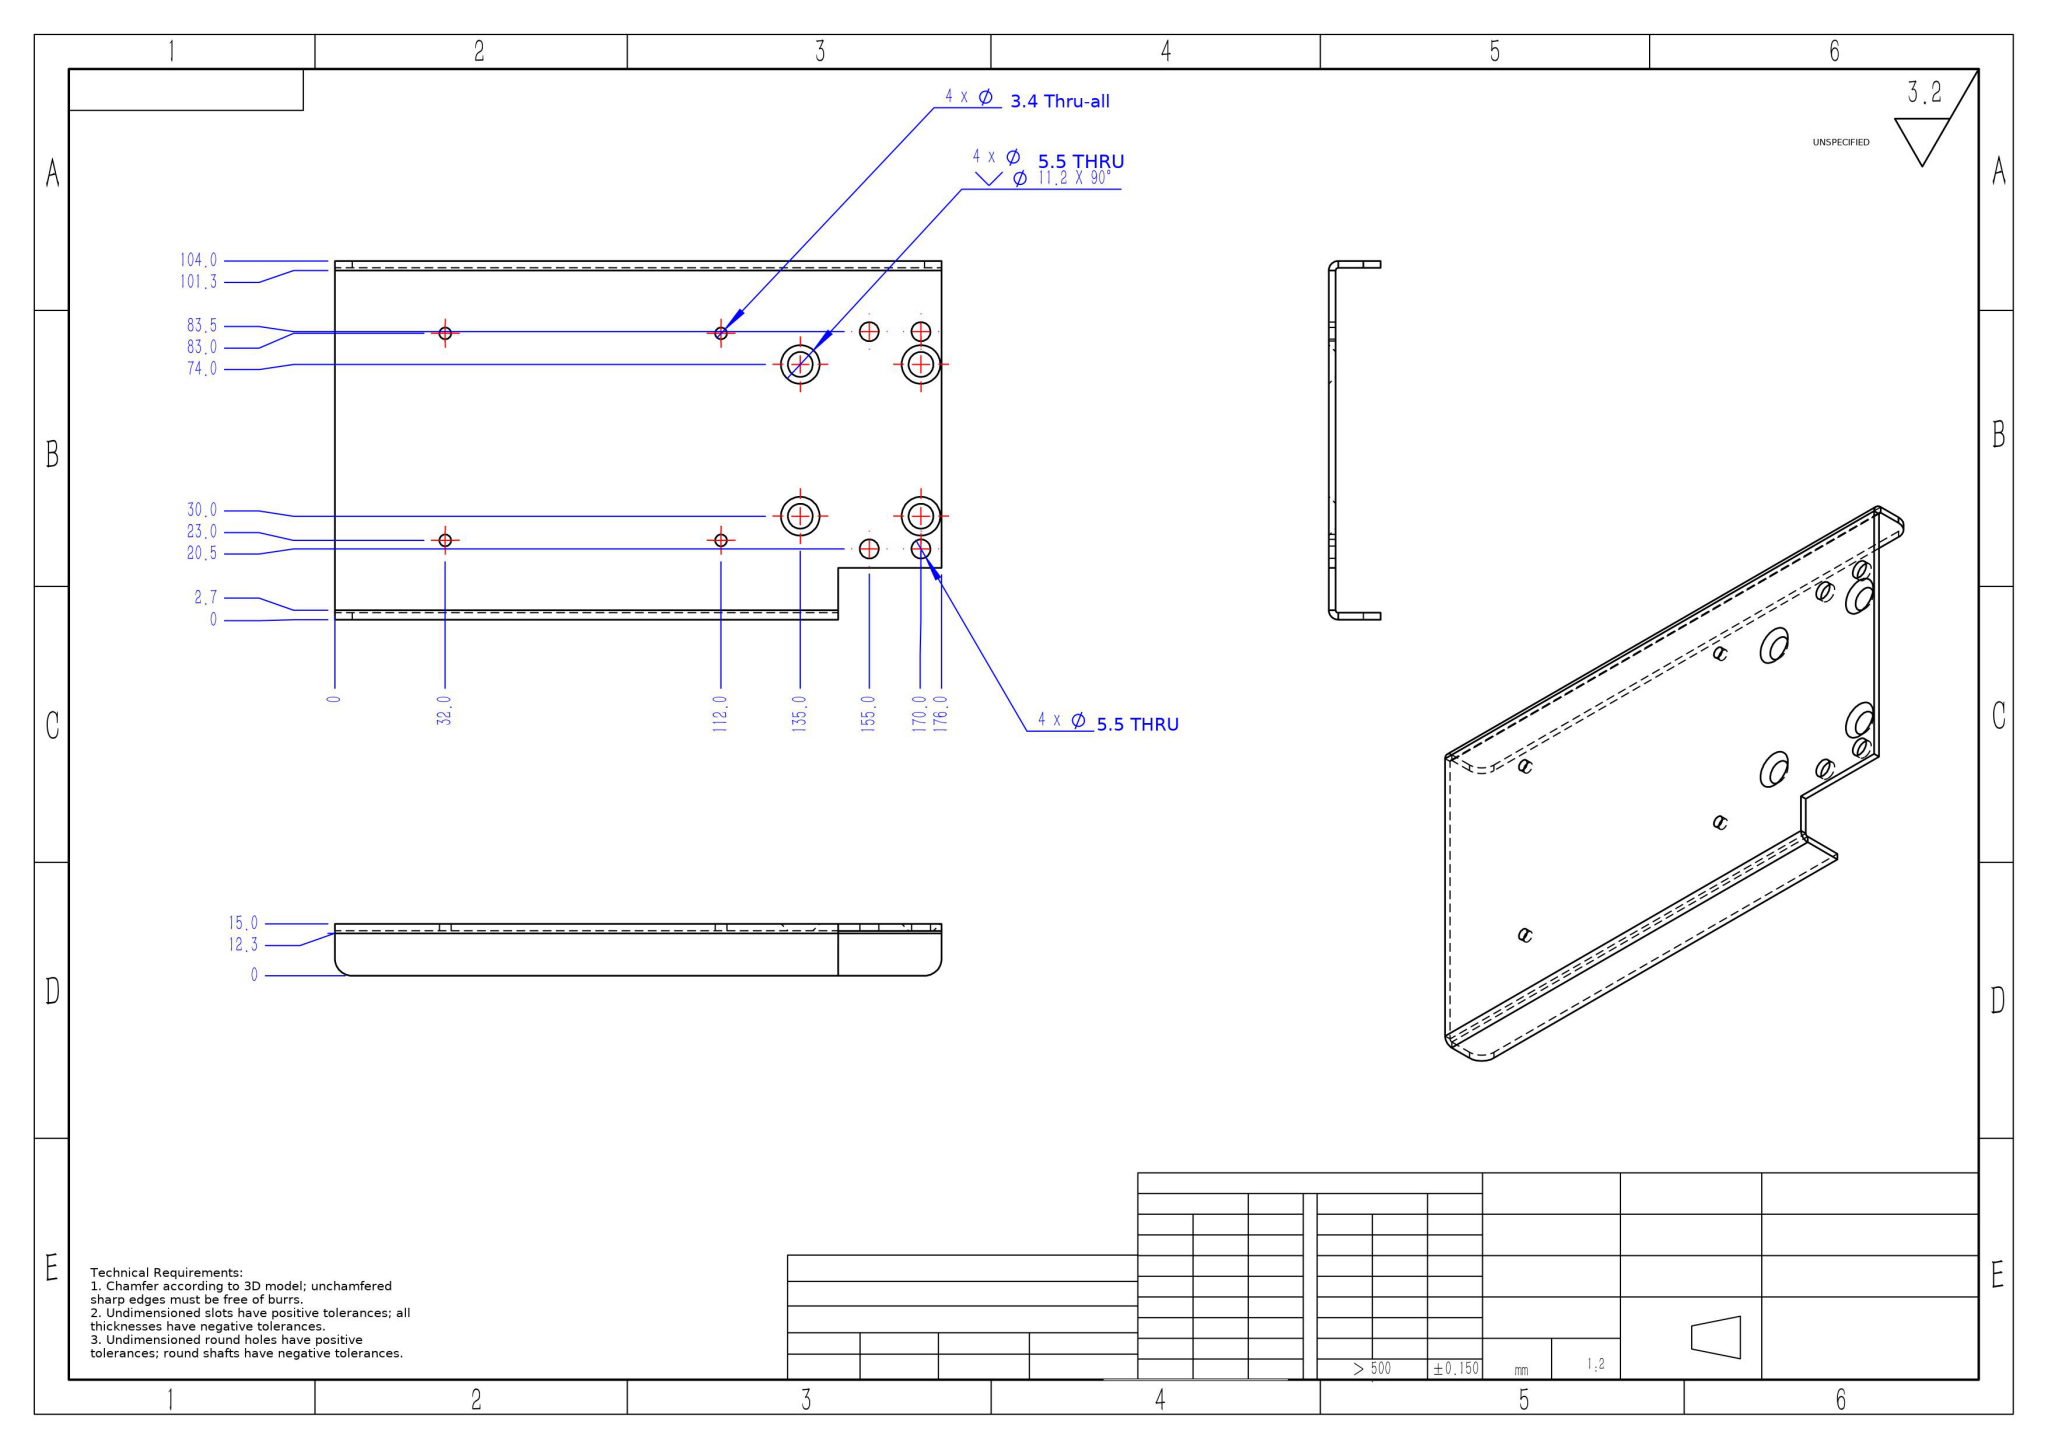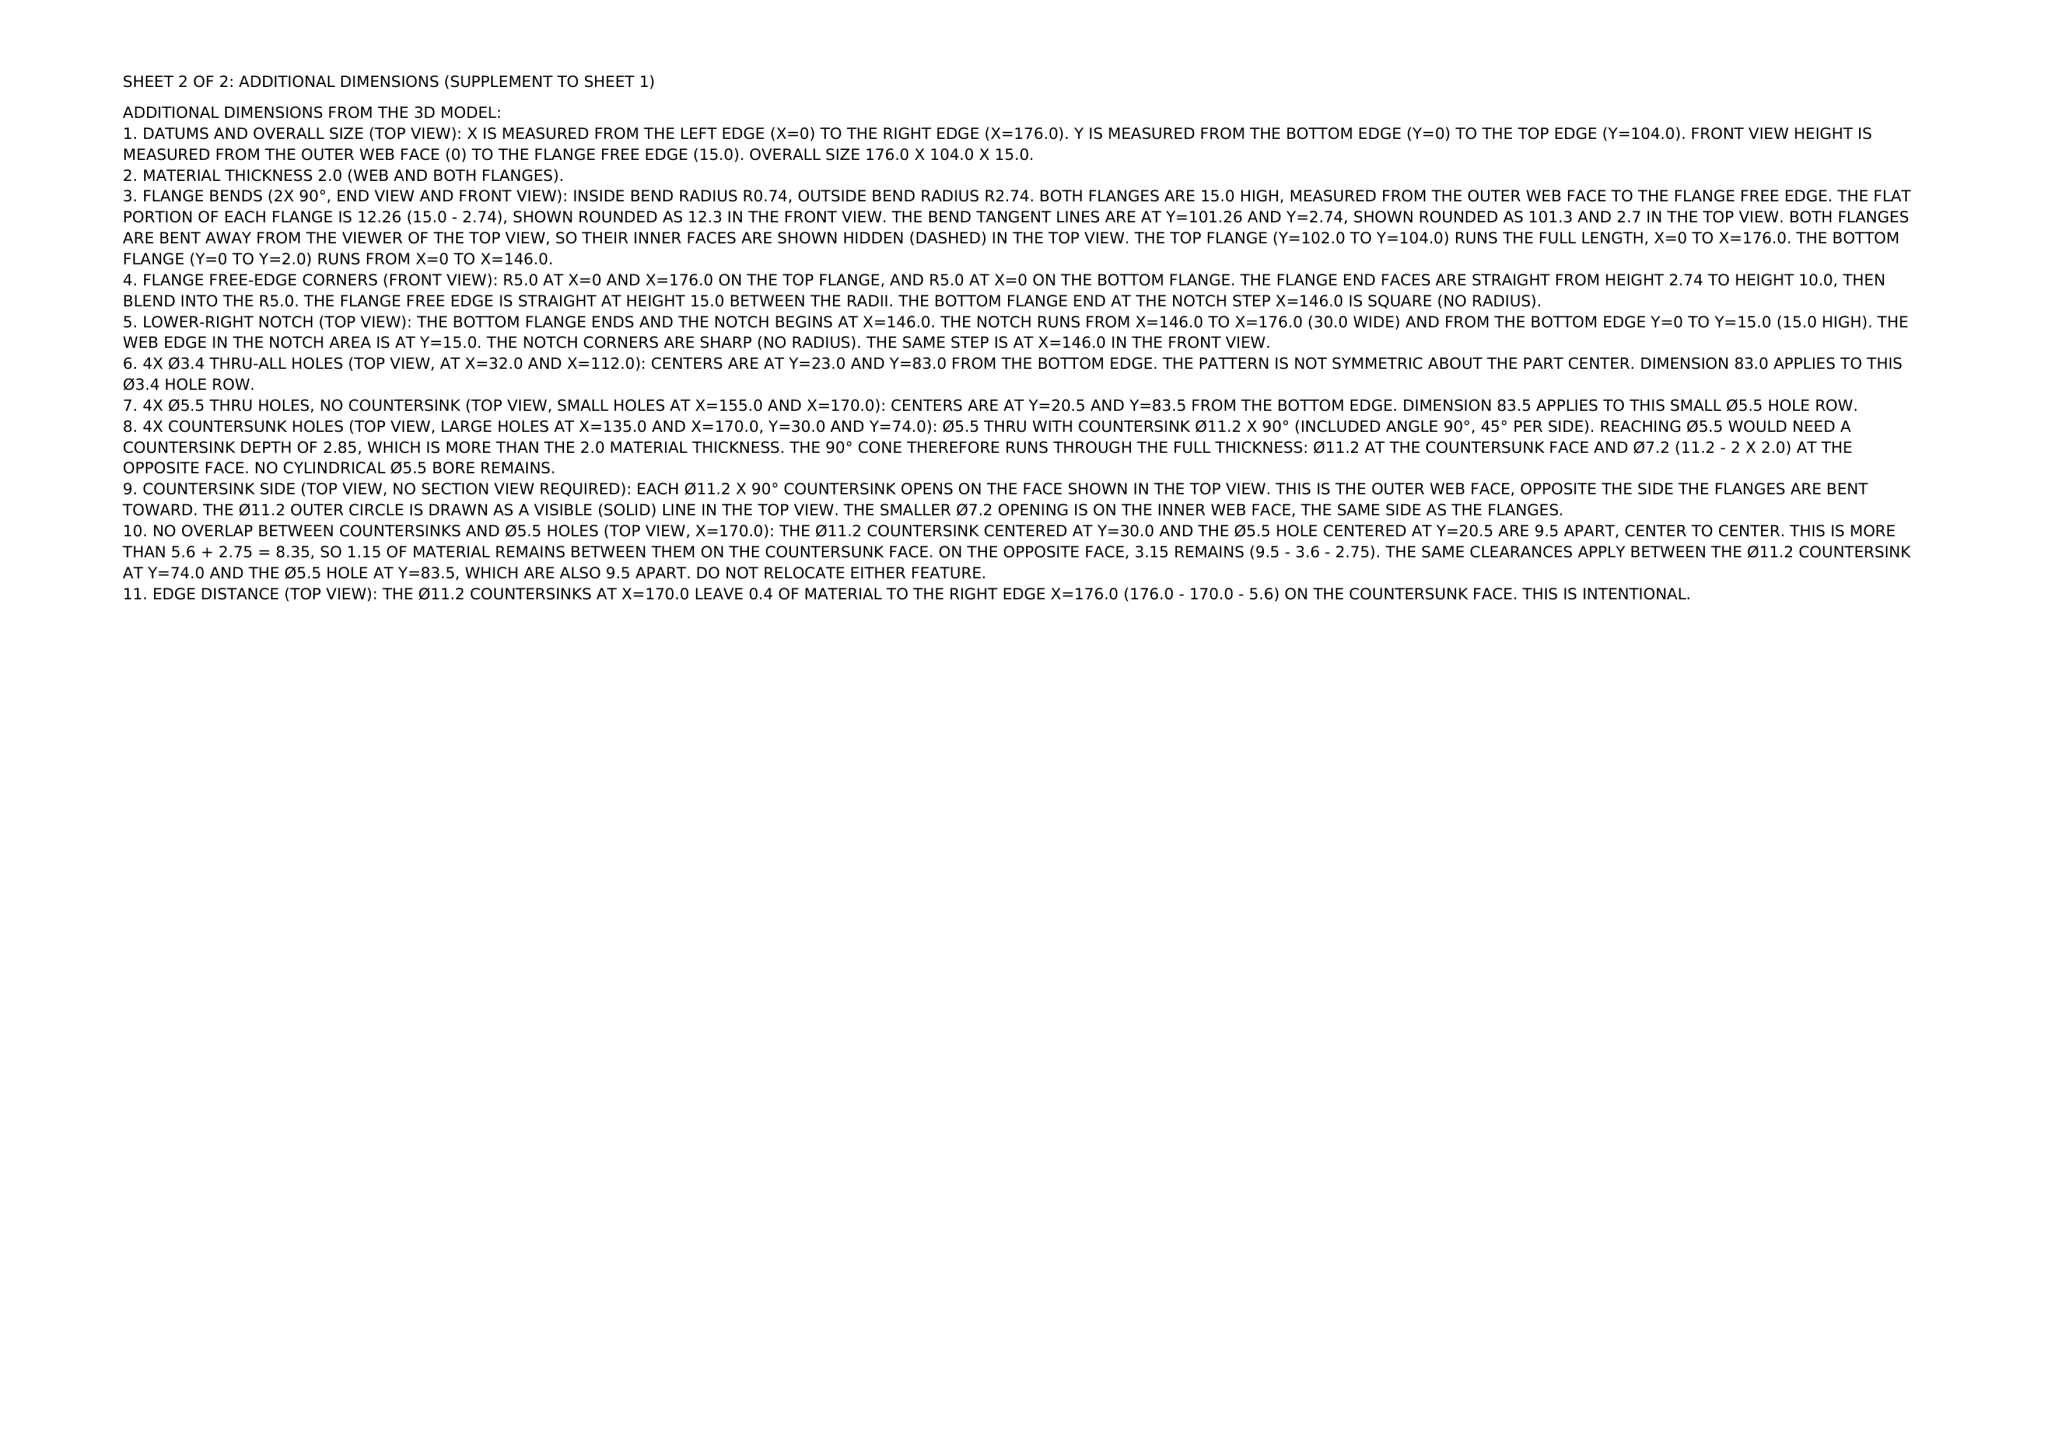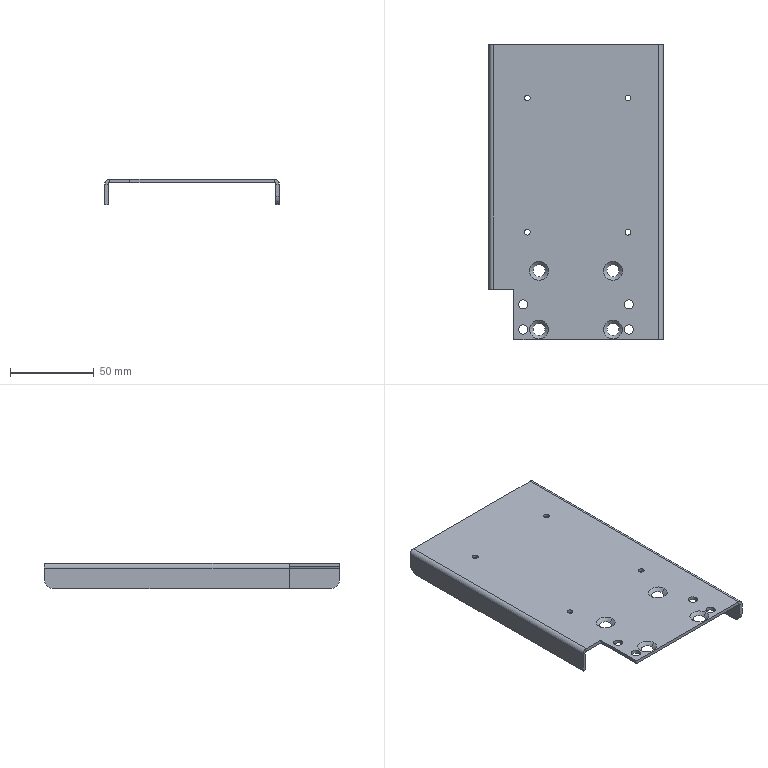Part | NX | mm | 1 solid | 51 faces | box 104 x 176 x 15 mm | volume 42765 mm3 | cylinder 23 | plane 20 | cone 8 | commonest cylinder face diameters 5.5 x8 3.4 x8 10 x3 5.473 x2 1.473 x2